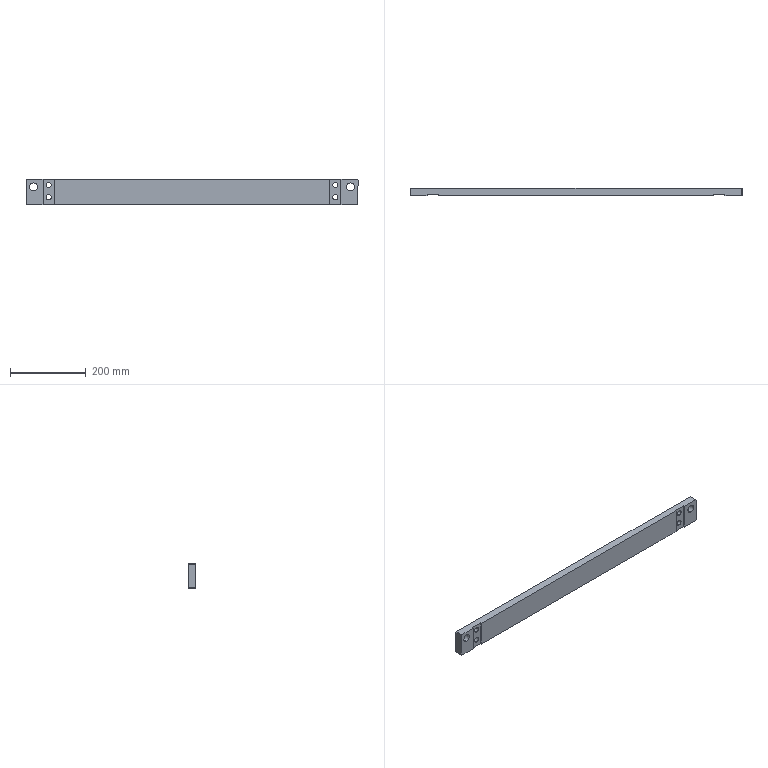Component | SolidWorks | FE2-211-_T_w_(-1 | 1 solid | 30 faces | box 878 x 20 x 67 mm | volume 1139978 mm3 | plane 18 | cylinder 12 | commonest cylinder face diameters 14 x8 21 x4
build123d program:
from build123d import *

# Parameters (mm, degrees)
SKETCH1_W      = 878
SKETCH1_H      = 67
EXTRUDE1_DEPTH = 20
SKETCH2_W      = 30
SKETCH2_H      = 67
EXTRUDE2_DEPTH = 3
SKETCH3_R      = 10.5
EXTRUDE3_DEPTH = 441.73
SKETCH4_R      = 7
EXTRUDE4_DEPTH = 441.604
CHAMFER1_SIZE  = 2


with BuildPart() as part:
    # Sketch1 → Extrude1 (new body)
    with BuildSketch(Plane(origin=(0, 0, 0), x_dir=(1, 0, 0), z_dir=(0, 1, 0))):
        Rectangle(SKETCH1_W, SKETCH1_H)
    extrude(amount=EXTRUDE1_DEPTH)

    # Sketch2 → Extrude2 (cut)
    with BuildSketch(Plane(origin=(0, 20, 0), x_dir=(1, 0, 0), z_dir=(0, 1, 0))):
        with Locations((379, 0)):
            Rectangle(SKETCH2_W, SKETCH2_H)
        with Locations((-379, 0)):
            Rectangle(SKETCH2_W, SKETCH2_H)
    extrude(amount=-EXTRUDE2_DEPTH, mode=Mode.SUBTRACT)

    # Sketch3 → Extrude3 (cut, through all)
    with BuildSketch(Plane(origin=(0, 20, 0), x_dir=(1, 0, 0), z_dir=(0, 1, 0))):
        with Locations(Location((419, 13.5, 0), (0, 0, 270))):
            Circle(SKETCH3_R)
        with Locations(Location((-419, 13.5, 0), (0, 0, 90))):
            Circle(SKETCH3_R)
    extrude(amount=-EXTRUDE3_DEPTH, mode=Mode.SUBTRACT)

    # Sketch4 → Extrude4 (cut, through all)
    with BuildSketch(Plane(origin=(0, 17, 0), x_dir=(1, 0, 0), z_dir=(0, 1, 0))):
        with Locations(Location((379, 18.5, 0), (0, 0, 270))):
            Circle(SKETCH4_R)
        with Locations(Location((379, -13.5, 0), (0, 0, 270))):
            Circle(SKETCH4_R)
        with Locations(Location((-379, -13.5, 0), (0, 0, 90))):
            Circle(SKETCH4_R)
        with Locations(Location((-379, 18.5, 0), (0, 0, 90))):
            Circle(SKETCH4_R)
    extrude(amount=-EXTRUDE4_DEPTH, mode=Mode.SUBTRACT)

    # Chamfer1
    chamfer1_edges = [part.edges().sort_by_distance(p)[0] for p in [
        (-439, 10, -33.5),
        (439, 10, -33.5),
        (439, 10, 33.5),
        (-439, 10, 33.5),
    ]]
    chamfer(chamfer1_edges, length=CHAMFER1_SIZE)


solid = part.part

# Placed as in the assembly
solid = solid.moved(Location((-379, 126.5, 311.5), (180, 0, 0)))
STEP:
#1=COLOUR_RGB('',0.7922,0.8196,0.9333);
#2=FILL_AREA_STYLE_COLOUR('',#1);
#3=FILL_AREA_STYLE('',(#2));
#4=SURFACE_STYLE_FILL_AREA(#3);
#5=SURFACE_SIDE_STYLE('',(#4));
#6=SURFACE_STYLE_USAGE(.BOTH.,#5);
#7=PRESENTATION_STYLE_ASSIGNMENT((#6));
#8=CARTESIAN_POINT('',(-29.843,4.98,13.268));
#9=VERTEX_POINT('',#8);
#10=CARTESIAN_POINT('',(-29.843,4.98,12.717));
#11=VERTEX_POINT('',#10);
#12=CARTESIAN_POINT('',(-29.843,4.98,12.992));
#13=DIRECTION('',(0.,-1.,0.));
#14=DIRECTION('',(0.,0.,1.));
#15=AXIS2_PLACEMENT_3D('',#12,#13,#14);
#16=CIRCLE('',#15,0.2756);
#17=EDGE_CURVE('',#9,#11,#16,.T.);
#18=ORIENTED_EDGE('',*,*,#17,.F.);
#19=CARTESIAN_POINT('',(-29.843,4.311,13.268));
#20=VERTEX_POINT('',#19);
#21=CARTESIAN_POINT('',(-29.843,4.98,13.268));
#22=DIRECTION('',(0.,-1.,0.));
#23=VECTOR('',#22,39.37);
#24=LINE('',#21,#23);
#25=EDGE_CURVE('',#9,#20,#24,.T.);
#26=ORIENTED_EDGE('',*,*,#25,.T.);
#27=CARTESIAN_POINT('',(-29.843,4.311,12.717));
#28=VERTEX_POINT('',#27);
#29=CARTESIAN_POINT('',(-29.843,4.311,12.992));
#30=DIRECTION('',(0.,-1.,0.));
#31=DIRECTION('',(0.,0.,1.));
#32=AXIS2_PLACEMENT_3D('',#29,#30,#31);
#33=CIRCLE('',#32,0.2756);
#34=EDGE_CURVE('',#20,#28,#33,.T.);
#35=ORIENTED_EDGE('',*,*,#34,.T.);
#36=CARTESIAN_POINT('',(-29.843,4.98,12.717));
#37=DIRECTION('',(0.,-1.,0.));
#38=VECTOR('',#37,39.37);
#39=LINE('',#36,#38);
#40=EDGE_CURVE('',#11,#28,#39,.T.);
#41=ORIENTED_EDGE('',*,*,#40,.F.);
#42=EDGE_LOOP('',(#18,#26,#35,#41));
#43=FACE_OUTER_BOUND('',#42,.T.);
#44=CARTESIAN_POINT('',(-29.843,4.98,12.992));
#45=DIRECTION('',(0.,-1.,0.));
#46=DIRECTION('',(0.,0.,-1.));
#47=AXIS2_PLACEMENT_3D('',#44,#45,#46);
#48=CYLINDRICAL_SURFACE('',#47,0.2756);
#49=ADVANCED_FACE('',(#43),#48,.F.);
#50=CARTESIAN_POINT('',(-29.843,4.98,12.008));
#51=VERTEX_POINT('',#50);
#52=CARTESIAN_POINT('',(-29.843,4.98,11.457));
#53=VERTEX_POINT('',#52);
#54=CARTESIAN_POINT('',(-29.843,4.98,11.732));
#55=DIRECTION('',(0.,-1.,0.));
#56=DIRECTION('',(0.,0.,1.));
#57=AXIS2_PLACEMENT_3D('',#54,#55,#56);
#58=CIRCLE('',#57,0.2756);
#59=EDGE_CURVE('',#51,#53,#58,.T.);
#60=ORIENTED_EDGE('',*,*,#59,.F.);
#61=CARTESIAN_POINT('',(-29.843,4.311,12.008));
#62=VERTEX_POINT('',#61);
#63=CARTESIAN_POINT('',(-29.843,4.98,12.008));
#64=DIRECTION('',(0.,-1.,0.));
#65=VECTOR('',#64,39.37);
#66=LINE('',#63,#65);
#67=EDGE_CURVE('',#51,#62,#66,.T.);
#68=ORIENTED_EDGE('',*,*,#67,.T.);
#69=CARTESIAN_POINT('',(-29.843,4.311,11.457));
#70=VERTEX_POINT('',#69);
#71=CARTESIAN_POINT('',(-29.843,4.311,11.732));
#72=DIRECTION('',(0.,-1.,0.));
#73=DIRECTION('',(0.,0.,1.));
#74=AXIS2_PLACEMENT_3D('',#71,#72,#73);
#75=CIRCLE('',#74,0.2756);
#76=EDGE_CURVE('',#62,#70,#75,.T.);
#77=ORIENTED_EDGE('',*,*,#76,.T.);
#78=CARTESIAN_POINT('',(-29.843,4.98,11.457));
#79=DIRECTION('',(0.,-1.,0.));
#80=VECTOR('',#79,39.37);
#81=LINE('',#78,#80);
#82=EDGE_CURVE('',#53,#70,#81,.T.);
#83=ORIENTED_EDGE('',*,*,#82,.F.);
#84=EDGE_LOOP('',(#60,#68,#77,#83));
#85=FACE_OUTER_BOUND('',#84,.T.);
#86=CARTESIAN_POINT('',(-29.843,4.98,11.732));
#87=DIRECTION('',(0.,-1.,0.));
#88=DIRECTION('',(0.,0.,-1.));
#89=AXIS2_PLACEMENT_3D('',#86,#87,#88);
#90=CYLINDRICAL_SURFACE('',#89,0.2756);
#91=ADVANCED_FACE('',(#85),#90,.F.);
#92=CARTESIAN_POINT('',(0.,4.98,12.008));
#93=VERTEX_POINT('',#92);
#94=CARTESIAN_POINT('',(0.,4.98,11.457));
#95=VERTEX_POINT('',#94);
#96=CARTESIAN_POINT('',(0.,4.98,11.732));
#97=DIRECTION('',(0.,-1.,0.));
#98=DIRECTION('',(-0.,0.,-1.));
#99=AXIS2_PLACEMENT_3D('',#96,#97,#98);
#100=CIRCLE('',#99,0.2756);
#101=EDGE_CURVE('',#93,#95,#100,.T.);
#102=ORIENTED_EDGE('',*,*,#101,.F.);
#103=CARTESIAN_POINT('',(0.,4.311,12.008));
#104=VERTEX_POINT('',#103);
#105=CARTESIAN_POINT('',(0.,4.98,12.008));
#106=DIRECTION('',(0.,-1.,0.));
#107=VECTOR('',#106,39.37);
#108=LINE('',#105,#107);
#109=EDGE_CURVE('',#93,#104,#108,.T.);
#110=ORIENTED_EDGE('',*,*,#109,.T.);
#111=CARTESIAN_POINT('',(0.,4.311,11.457));
#112=VERTEX_POINT('',#111);
#113=CARTESIAN_POINT('',(0.,4.311,11.732));
#114=DIRECTION('',(0.,-1.,0.));
#115=DIRECTION('',(-0.,0.,-1.));
#116=AXIS2_PLACEMENT_3D('',#113,#114,#115);
#117=CIRCLE('',#116,0.2756);
#118=EDGE_CURVE('',#104,#112,#117,.T.);
#119=ORIENTED_EDGE('',*,*,#118,.T.);
#120=CARTESIAN_POINT('',(0.,4.98,11.457));
#121=DIRECTION('',(0.,-1.,0.));
#122=VECTOR('',#121,39.37);
#123=LINE('',#120,#122);
#124=EDGE_CURVE('',#95,#112,#123,.T.);
#125=ORIENTED_EDGE('',*,*,#124,.F.);
#126=EDGE_LOOP('',(#102,#110,#119,#125));
#127=FACE_OUTER_BOUND('',#126,.T.);
#128=CARTESIAN_POINT('',(0.,4.98,11.732));
#129=DIRECTION('',(0.,-1.,0.));
#130=DIRECTION('',(-0.,0.,-1.));
#131=AXIS2_PLACEMENT_3D('',#128,#129,#130);
#132=CYLINDRICAL_SURFACE('',#131,0.2756);
#133=ADVANCED_FACE('',(#127),#132,.F.);
#134=CARTESIAN_POINT('',(0.,4.98,13.268));
#135=VERTEX_POINT('',#134);
#136=CARTESIAN_POINT('',(0.,4.98,12.717));
#137=VERTEX_POINT('',#136);
#138=CARTESIAN_POINT('',(0.,4.98,12.992));
#139=DIRECTION('',(0.,-1.,0.));
#140=DIRECTION('',(-0.,0.,-1.));
#141=AXIS2_PLACEMENT_3D('',#138,#139,#140);
#142=CIRCLE('',#141,0.2756);
#143=EDGE_CURVE('',#135,#137,#142,.T.);
#144=ORIENTED_EDGE('',*,*,#143,.F.);
#145=CARTESIAN_POINT('',(0.,4.311,13.268));
#146=VERTEX_POINT('',#145);
#147=CARTESIAN_POINT('',(0.,4.98,13.268));
#148=DIRECTION('',(0.,-1.,0.));
#149=VECTOR('',#148,39.37);
#150=LINE('',#147,#149);
#151=EDGE_CURVE('',#135,#146,#150,.T.);
#152=ORIENTED_EDGE('',*,*,#151,.T.);
#153=CARTESIAN_POINT('',(0.,4.311,12.717));
#154=VERTEX_POINT('',#153);
#155=CARTESIAN_POINT('',(0.,4.311,12.992));
#156=DIRECTION('',(0.,-1.,0.));
#157=DIRECTION('',(-0.,0.,-1.));
#158=AXIS2_PLACEMENT_3D('',#155,#156,#157);
#159=CIRCLE('',#158,0.2756);
#160=EDGE_CURVE('',#146,#154,#159,.T.);
#161=ORIENTED_EDGE('',*,*,#160,.T.);
#162=CARTESIAN_POINT('',(0.,4.98,12.717));
#163=DIRECTION('',(0.,-1.,0.));
#164=VECTOR('',#163,39.37);
#165=LINE('',#162,#164);
#166=EDGE_CURVE('',#137,#154,#165,.T.);
#167=ORIENTED_EDGE('',*,*,#166,.F.);
#168=EDGE_LOOP('',(#144,#152,#161,#167));
#169=FACE_OUTER_BOUND('',#168,.T.);
#170=CARTESIAN_POINT('',(0.,4.98,12.992));
#171=DIRECTION('',(0.,-1.,0.));
#172=DIRECTION('',(-0.,0.,-1.));
#173=AXIS2_PLACEMENT_3D('',#170,#171,#172);
#174=CYLINDRICAL_SURFACE('',#173,0.2756);
#175=ADVANCED_FACE('',(#169),#174,.F.);
#176=CARTESIAN_POINT('',(-31.417,4.98,13.209));
#177=VERTEX_POINT('',#176);
#178=CARTESIAN_POINT('',(-31.417,4.98,12.382));
#179=VERTEX_POINT('',#178);
#180=CARTESIAN_POINT('',(-31.417,4.98,12.795));
#181=DIRECTION('',(0.,-1.,0.));
#182=DIRECTION('',(0.,0.,1.));
#183=AXIS2_PLACEMENT_3D('',#180,#181,#182);
#184=CIRCLE('',#183,0.4134);
#185=EDGE_CURVE('',#177,#179,#184,.T.);
#186=ORIENTED_EDGE('',*,*,#185,.F.);
#187=CARTESIAN_POINT('',(-31.417,4.193,13.209));
#188=VERTEX_POINT('',#187);
#189=CARTESIAN_POINT('',(-31.417,4.98,13.209));
#190=DIRECTION('',(0.,-1.,0.));
#191=VECTOR('',#190,39.37);
#192=LINE('',#189,#191);
#193=EDGE_CURVE('',#177,#188,#192,.T.);
#194=ORIENTED_EDGE('',*,*,#193,.T.);
#195=CARTESIAN_POINT('',(-31.417,4.193,12.382));
#196=VERTEX_POINT('',#195);
#197=CARTESIAN_POINT('',(-31.417,4.193,12.795));
#198=DIRECTION('',(0.,-1.,0.));
#199=DIRECTION('',(0.,0.,1.));
#200=AXIS2_PLACEMENT_3D('',#197,#198,#199);
#201=CIRCLE('',#200,0.4134);
#202=EDGE_CURVE('',#188,#196,#201,.T.);
#203=ORIENTED_EDGE('',*,*,#202,.T.);
#204=CARTESIAN_POINT('',(-31.417,4.98,12.382));
#205=DIRECTION('',(0.,-1.,0.));
#206=VECTOR('',#205,39.37);
#207=LINE('',#204,#206);
#208=EDGE_CURVE('',#179,#196,#207,.T.);
#209=ORIENTED_EDGE('',*,*,#208,.F.);
#210=EDGE_LOOP('',(#186,#194,#203,#209));
#211=FACE_OUTER_BOUND('',#210,.T.);
#212=CARTESIAN_POINT('',(-31.417,4.98,12.795));
#213=DIRECTION('',(0.,-1.,0.));
#214=DIRECTION('',(0.,0.,-1.));
#215=AXIS2_PLACEMENT_3D('',#212,#213,#214);
#216=CYLINDRICAL_SURFACE('',#215,0.4134);
#217=ADVANCED_FACE('',(#211),#216,.F.);
#218=CARTESIAN_POINT('',(1.575,4.98,13.209));
#219=VERTEX_POINT('',#218);
#220=CARTESIAN_POINT('',(1.575,4.98,12.382));
#221=VERTEX_POINT('',#220);
#222=CARTESIAN_POINT('',(1.575,4.98,12.795));
#223=DIRECTION('',(0.,-1.,0.));
#224=DIRECTION('',(-0.,0.,-1.));
#225=AXIS2_PLACEMENT_3D('',#222,#223,#224);
#226=CIRCLE('',#225,0.4134);
#227=EDGE_CURVE('',#219,#221,#226,.T.);
#228=ORIENTED_EDGE('',*,*,#227,.F.);
#229=CARTESIAN_POINT('',(1.575,4.193,13.209));
#230=VERTEX_POINT('',#229);
#231=CARTESIAN_POINT('',(1.575,4.98,13.209));
#232=DIRECTION('',(0.,-1.,0.));
#233=VECTOR('',#232,39.37);
#234=LINE('',#231,#233);
#235=EDGE_CURVE('',#219,#230,#234,.T.);
#236=ORIENTED_EDGE('',*,*,#235,.T.);
#237=CARTESIAN_POINT('',(1.575,4.193,12.382));
#238=VERTEX_POINT('',#237);
#239=CARTESIAN_POINT('',(1.575,4.193,12.795));
#240=DIRECTION('',(0.,-1.,0.));
#241=DIRECTION('',(-0.,0.,-1.));
#242=AXIS2_PLACEMENT_3D('',#239,#240,#241);
#243=CIRCLE('',#242,0.4134);
#244=EDGE_CURVE('',#230,#238,#243,.T.);
#245=ORIENTED_EDGE('',*,*,#244,.T.);
#246=CARTESIAN_POINT('',(1.575,4.98,12.382));
#247=DIRECTION('',(0.,-1.,0.));
#248=VECTOR('',#247,39.37);
#249=LINE('',#246,#248);
#250=EDGE_CURVE('',#221,#238,#249,.T.);
#251=ORIENTED_EDGE('',*,*,#250,.F.);
#252=EDGE_LOOP('',(#228,#236,#245,#251));
#253=FACE_OUTER_BOUND('',#252,.T.);
#254=CARTESIAN_POINT('',(1.575,4.98,12.795));
#255=DIRECTION('',(0.,-1.,0.));
#256=DIRECTION('',(-0.,0.,-1.));
#257=AXIS2_PLACEMENT_3D('',#254,#255,#256);
#258=CYLINDRICAL_SURFACE('',#257,0.4134);
#259=ADVANCED_FACE('',(#253),#258,.F.);
#260=CARTESIAN_POINT('',(-29.252,4.193,10.945));
#261=VERTEX_POINT('',#260);
#262=CARTESIAN_POINT('',(-29.252,4.193,13.583));
#263=VERTEX_POINT('',#262);
#264=CARTESIAN_POINT('',(-29.252,4.193,13.583));
#265=DIRECTION('',(0.,0.,1.));
#266=VECTOR('',#265,39.37);
#267=LINE('',#264,#266);
#268=EDGE_CURVE('',#261,#263,#267,.T.);
#269=ORIENTED_EDGE('',*,*,#268,.F.);
#270=CARTESIAN_POINT('',(-0.5906,4.193,10.945));
#271=VERTEX_POINT('',#270);
#272=CARTESIAN_POINT('',(2.362,4.193,10.945));
#273=DIRECTION('',(1.,0.,-0.));
#274=VECTOR('',#273,39.37);
#275=LINE('',#272,#274);
#276=EDGE_CURVE('',#261,#271,#275,.T.);
#277=ORIENTED_EDGE('',*,*,#276,.T.);
#278=CARTESIAN_POINT('',(-0.5906,4.193,13.583));
#279=VERTEX_POINT('',#278);
#280=CARTESIAN_POINT('',(-0.5906,4.193,13.583));
#281=DIRECTION('',(-0.,0.,-1.));
#282=VECTOR('',#281,39.37);
#283=LINE('',#280,#282);
#284=EDGE_CURVE('',#279,#271,#283,.T.);
#285=ORIENTED_EDGE('',*,*,#284,.F.);
#286=CARTESIAN_POINT('',(2.362,4.193,13.583));
#287=DIRECTION('',(-1.,0.,0.));
#288=VECTOR('',#287,39.37);
#289=LINE('',#286,#288);
#290=EDGE_CURVE('',#279,#263,#289,.T.);
#291=ORIENTED_EDGE('',*,*,#290,.T.);
#292=EDGE_LOOP('',(#269,#277,#285,#291));
#293=FACE_OUTER_BOUND('',#292,.T.);
#294=CARTESIAN_POINT('',(-32.205,4.193,13.583));
#295=DIRECTION('',(0.,-1.,0.));
#296=DIRECTION('',(-0.,0.,-1.));
#297=AXIS2_PLACEMENT_3D('',#294,#295,#296);
#298=PLANE('',#297);
#299=ADVANCED_FACE('',(#293),#298,.T.);
#300=CARTESIAN_POINT('',(-31.417,4.193,12.795));
#301=DIRECTION('',(0.,-1.,0.));
#302=DIRECTION('',(0.,0.,1.));
#303=AXIS2_PLACEMENT_3D('',#300,#301,#302);
#304=CIRCLE('',#303,0.4134);
#305=EDGE_CURVE('',#196,#188,#304,.T.);
#306=ORIENTED_EDGE('',*,*,#305,.F.);
#307=ORIENTED_EDGE('',*,*,#202,.F.);
#308=EDGE_LOOP('',(#306,#307));
#309=FACE_BOUND('',#308,.T.);
#310=CARTESIAN_POINT('',(-30.433,4.193,13.583));
#311=VERTEX_POINT('',#310);
#312=CARTESIAN_POINT('',(-32.126,4.193,13.583));
#313=VERTEX_POINT('',#312);
#314=CARTESIAN_POINT('',(2.362,4.193,13.583));
#315=DIRECTION('',(-1.,0.,0.));
#316=VECTOR('',#315,39.37);
#317=LINE('',#314,#316);
#318=EDGE_CURVE('',#311,#313,#317,.T.);
#319=ORIENTED_EDGE('',*,*,#318,.T.);
#320=CARTESIAN_POINT('',(-32.205,4.193,13.504));
#321=VERTEX_POINT('',#320);
#322=CARTESIAN_POINT('',(-32.165,4.193,13.543));
#323=DIRECTION('',(-0.7071,0.,-0.7071));
#324=VECTOR('',#323,39.37);
#325=LINE('',#322,#324);
#326=EDGE_CURVE('',#313,#321,#325,.T.);
#327=ORIENTED_EDGE('',*,*,#326,.T.);
#328=CARTESIAN_POINT('',(-32.205,4.193,11.024));
#329=VERTEX_POINT('',#328);
#330=CARTESIAN_POINT('',(-32.205,4.193,10.945));
#331=DIRECTION('',(-0.,0.,-1.));
#332=VECTOR('',#331,39.37);
#333=LINE('',#330,#332);
#334=EDGE_CURVE('',#321,#329,#333,.T.);
#335=ORIENTED_EDGE('',*,*,#334,.T.);
#336=CARTESIAN_POINT('',(-32.126,4.193,10.945));
#337=VERTEX_POINT('',#336);
#338=CARTESIAN_POINT('',(-33.484,4.193,12.303));
#339=DIRECTION('',(0.7071,0.,-0.7071));
#340=VECTOR('',#339,39.37);
#341=LINE('',#338,#340);
#342=EDGE_CURVE('',#329,#337,#341,.T.);
#343=ORIENTED_EDGE('',*,*,#342,.T.);
#344=CARTESIAN_POINT('',(-30.433,4.193,10.945));
#345=VERTEX_POINT('',#344);
#346=CARTESIAN_POINT('',(2.362,4.193,10.945));
#347=DIRECTION('',(1.,0.,-0.));
#348=VECTOR('',#347,39.37);
#349=LINE('',#346,#348);
#350=EDGE_CURVE('',#337,#345,#349,.T.);
#351=ORIENTED_EDGE('',*,*,#350,.T.);
#352=CARTESIAN_POINT('',(-30.433,4.193,13.583));
#353=DIRECTION('',(-0.,0.,-1.));
#354=VECTOR('',#353,39.37);
#355=LINE('',#352,#354);
#356=EDGE_CURVE('',#311,#345,#355,.T.);
#357=ORIENTED_EDGE('',*,*,#356,.F.);
#358=EDGE_LOOP('',(#319,#327,#335,#343,#351,#357));
#359=FACE_OUTER_BOUND('',#358,.T.);
#360=CARTESIAN_POINT('',(-32.205,4.193,13.583));
#361=DIRECTION('',(0.,-1.,0.));
#362=DIRECTION('',(-0.,0.,-1.));
#363=AXIS2_PLACEMENT_3D('',#360,#361,#362);
#364=PLANE('',#363);
#365=ADVANCED_FACE('',(#309,#359),#364,.T.);
#366=ORIENTED_EDGE('',*,*,#334,.F.);
#367=CARTESIAN_POINT('',(-32.205,4.98,13.504));
#368=VERTEX_POINT('',#367);
#369=CARTESIAN_POINT('',(-32.205,4.193,13.504));
#370=DIRECTION('',(0.,1.,0.));
#371=VECTOR('',#370,39.37);
#372=LINE('',#369,#371);
#373=EDGE_CURVE('',#321,#368,#372,.T.);
#374=ORIENTED_EDGE('',*,*,#373,.T.);
#375=CARTESIAN_POINT('',(-32.205,4.98,11.024));
#376=VERTEX_POINT('',#375);
#377=CARTESIAN_POINT('',(-32.205,4.98,10.945));
#378=DIRECTION('',(-0.,0.,-1.));
#379=VECTOR('',#378,39.37);
#380=LINE('',#377,#379);
#381=EDGE_CURVE('',#368,#376,#380,.T.);
#382=ORIENTED_EDGE('',*,*,#381,.T.);
#383=CARTESIAN_POINT('',(-32.205,4.193,11.024));
#384=DIRECTION('',(0.,-1.,0.));
#385=VECTOR('',#384,39.37);
#386=LINE('',#383,#385);
#387=EDGE_CURVE('',#376,#329,#386,.T.);
#388=ORIENTED_EDGE('',*,*,#387,.T.);
#389=EDGE_LOOP('',(#366,#374,#382,#388));
#390=FACE_OUTER_BOUND('',#389,.T.);
#391=CARTESIAN_POINT('',(-32.205,4.193,10.945));
#392=DIRECTION('',(1.,0.,-0.));
#393=DIRECTION('',(0.,0.,1.));
#394=AXIS2_PLACEMENT_3D('',#391,#392,#393);
#395=PLANE('',#394);
#396=ADVANCED_FACE('',(#390),#395,.F.);
#397=CARTESIAN_POINT('',(-32.126,4.98,10.945));
#398=VERTEX_POINT('',#397);
#399=CARTESIAN_POINT('',(2.283,4.98,10.945));
#400=VERTEX_POINT('',#399);
#401=CARTESIAN_POINT('',(2.362,4.98,10.945));
#402=DIRECTION('',(1.,0.,-0.));
#403=VECTOR('',#402,39.37);
#404=LINE('',#401,#403);
#405=EDGE_CURVE('',#398,#400,#404,.T.);
#406=ORIENTED_EDGE('',*,*,#405,.T.);
#407=CARTESIAN_POINT('',(2.283,4.193,10.945));
#408=VERTEX_POINT('',#407);
#409=CARTESIAN_POINT('',(2.283,4.193,10.945));
#410=DIRECTION('',(0.,-1.,0.));
#411=VECTOR('',#410,39.37);
#412=LINE('',#409,#411);
#413=EDGE_CURVE('',#400,#408,#412,.T.);
#414=ORIENTED_EDGE('',*,*,#413,.T.);
#415=CARTESIAN_POINT('',(0.5906,4.193,10.945));
#416=VERTEX_POINT('',#415);
#417=CARTESIAN_POINT('',(2.362,4.193,10.945));
#418=DIRECTION('',(1.,0.,-0.));
#419=VECTOR('',#418,39.37);
#420=LINE('',#417,#419);
#421=EDGE_CURVE('',#416,#408,#420,.T.);
#422=ORIENTED_EDGE('',*,*,#421,.F.);
#423=CARTESIAN_POINT('',(0.5906,4.311,10.945));
#424=VERTEX_POINT('',#423);
#425=CARTESIAN_POINT('',(0.5906,4.311,10.945));
#426=DIRECTION('',(0.,-1.,0.));
#427=VECTOR('',#426,39.37);
#428=LINE('',#425,#427);
#429=EDGE_CURVE('',#424,#416,#428,.T.);
#430=ORIENTED_EDGE('',*,*,#429,.F.);
#431=CARTESIAN_POINT('',(-0.5906,4.311,10.945));
#432=VERTEX_POINT('',#431);
#433=CARTESIAN_POINT('',(-0.5906,4.311,10.945));
#434=DIRECTION('',(1.,0.,-0.));
#435=VECTOR('',#434,39.37);
#436=LINE('',#433,#435);
#437=EDGE_CURVE('',#432,#424,#436,.T.);
#438=ORIENTED_EDGE('',*,*,#437,.F.);
#439=CARTESIAN_POINT('',(-0.5906,4.311,10.945));
#440=DIRECTION('',(0.,-1.,0.));
#441=VECTOR('',#440,39.37);
#442=LINE('',#439,#441);
#443=EDGE_CURVE('',#432,#271,#442,.T.);
#444=ORIENTED_EDGE('',*,*,#443,.T.);
#445=ORIENTED_EDGE('',*,*,#276,.F.);
#446=CARTESIAN_POINT('',(-29.252,4.311,10.945));
#447=VERTEX_POINT('',#446);
#448=CARTESIAN_POINT('',(-29.252,4.311,10.945));
#449=DIRECTION('',(0.,-1.,0.));
#450=VECTOR('',#449,39.37);
#451=LINE('',#448,#450);
#452=EDGE_CURVE('',#447,#261,#451,.T.);
#453=ORIENTED_EDGE('',*,*,#452,.F.);
#454=CARTESIAN_POINT('',(-30.433,4.311,10.945));
#455=VERTEX_POINT('',#454);
#456=CARTESIAN_POINT('',(-29.252,4.311,10.945));
#457=DIRECTION('',(1.,0.,-0.));
#458=VECTOR('',#457,39.37);
#459=LINE('',#456,#458);
#460=EDGE_CURVE('',#455,#447,#459,.T.);
#461=ORIENTED_EDGE('',*,*,#460,.F.);
#462=CARTESIAN_POINT('',(-30.433,4.311,10.945));
#463=DIRECTION('',(0.,-1.,0.));
#464=VECTOR('',#463,39.37);
#465=LINE('',#462,#464);
#466=EDGE_CURVE('',#455,#345,#465,.T.);
#467=ORIENTED_EDGE('',*,*,#466,.T.);
#468=ORIENTED_EDGE('',*,*,#350,.F.);
#469=CARTESIAN_POINT('',(-32.126,4.193,10.945));
#470=DIRECTION('',(0.,1.,0.));
#471=VECTOR('',#470,39.37);
#472=LINE('',#469,#471);
#473=EDGE_CURVE('',#337,#398,#472,.T.);
#474=ORIENTED_EDGE('',*,*,#473,.T.);
#475=EDGE_LOOP('',(#406,#414,#422,#430,#438,#444,#445,#453,#461,#467,#468,#474));
#476=FACE_OUTER_BOUND('',#475,.T.);
#477=CARTESIAN_POINT('',(2.362,4.193,10.945));
#478=DIRECTION('',(0.,0.,1.));
#479=DIRECTION('',(-1.,0.,0.));
#480=AXIS2_PLACEMENT_3D('',#477,#478,#479);
#481=PLANE('',#480);
#482=ADVANCED_FACE('',(#476),#481,.F.);
#483=CARTESIAN_POINT('',(2.362,4.98,11.024));
#484=VERTEX_POINT('',#483);
#485=CARTESIAN_POINT('',(2.362,4.98,13.504));
#486=VERTEX_POINT('',#485);
#487=CARTESIAN_POINT('',(2.362,4.98,10.945));
#488=DIRECTION('',(0.,0.,1.));
#489=VECTOR('',#488,39.37);
#490=LINE('',#487,#489);
#491=EDGE_CURVE('',#484,#486,#490,.T.);
#492=ORIENTED_EDGE('',*,*,#491,.T.);
#493=CARTESIAN_POINT('',(2.362,4.193,13.504));
#494=VERTEX_POINT('',#493);
#495=CARTESIAN_POINT('',(2.362,4.193,13.504));
#496=DIRECTION('',(0.,-1.,0.));
#497=VECTOR('',#496,39.37);
#498=LINE('',#495,#497);
#499=EDGE_CURVE('',#486,#494,#498,.T.);
#500=ORIENTED_EDGE('',*,*,#499,.T.);
#501=CARTESIAN_POINT('',(2.362,4.193,11.024));
#502=VERTEX_POINT('',#501);
#503=CARTESIAN_POINT('',(2.362,4.193,10.945));
#504=DIRECTION('',(0.,0.,1.));
#505=VECTOR('',#504,39.37);
#506=LINE('',#503,#505);
#507=EDGE_CURVE('',#502,#494,#506,.T.);
#508=ORIENTED_EDGE('',*,*,#507,.F.);
#509=CARTESIAN_POINT('',(2.362,4.193,11.024));
#510=DIRECTION('',(0.,1.,0.));
#511=VECTOR('',#510,39.37);
#512=LINE('',#509,#511);
#513=EDGE_CURVE('',#502,#484,#512,.T.);
#514=ORIENTED_EDGE('',*,*,#513,.T.);
#515=EDGE_LOOP('',(#492,#500,#508,#514));
#516=FACE_OUTER_BOUND('',#515,.T.);
#517=CARTESIAN_POINT('',(2.362,4.193,10.945));
#518=DIRECTION('',(-1.,0.,0.));
#519=DIRECTION('',(-0.,0.,-1.));
#520=AXIS2_PLACEMENT_3D('',#517,#518,#519);
#521=PLANE('',#520);
#522=ADVANCED_FACE('',(#516),#521,.F.);
#523=CARTESIAN_POINT('',(2.283,4.193,13.583));
#524=VERTEX_POINT('',#523);
#525=CARTESIAN_POINT('',(0.5906,4.193,13.583));
#526=VERTEX_POINT('',#525);
#527=CARTESIAN_POINT('',(2.362,4.193,13.583));
#528=DIRECTION('',(-1.,0.,0.));
#529=VECTOR('',#528,39.37);
#530=LINE('',#527,#529);
#531=EDGE_CURVE('',#524,#526,#530,.T.);
#532=ORIENTED_EDGE('',*,*,#531,.F.);
#533=CARTESIAN_POINT('',(2.283,4.98,13.583));
#534=VERTEX_POINT('',#533);
#535=CARTESIAN_POINT('',(2.283,4.193,13.583));
#536=DIRECTION('',(0.,1.,0.));
#537=VECTOR('',#536,39.37);
#538=LINE('',#535,#537);
#539=EDGE_CURVE('',#524,#534,#538,.T.);
#540=ORIENTED_EDGE('',*,*,#539,.T.);
#541=CARTESIAN_POINT('',(-32.126,4.98,13.583));
#542=VERTEX_POINT('',#541);
#543=CARTESIAN_POINT('',(2.362,4.98,13.583));
#544=DIRECTION('',(-1.,0.,0.));
#545=VECTOR('',#544,39.37);
#546=LINE('',#543,#545);
#547=EDGE_CURVE('',#534,#542,#546,.T.);
#548=ORIENTED_EDGE('',*,*,#547,.T.);
#549=CARTESIAN_POINT('',(-32.126,4.193,13.583));
#550=DIRECTION('',(0.,-1.,0.));
#551=VECTOR('',#550,39.37);
#552=LINE('',#549,#551);
#553=EDGE_CURVE('',#542,#313,#552,.T.);
#554=ORIENTED_EDGE('',*,*,#553,.T.);
#555=ORIENTED_EDGE('',*,*,#318,.F.);
#556=CARTESIAN_POINT('',(-30.433,4.311,13.583));
#557=VERTEX_POINT('',#556);
#558=CARTESIAN_POINT('',(-30.433,4.311,13.583));
#559=DIRECTION('',(0.,-1.,0.));
#560=VECTOR('',#559,39.37);
#561=LINE('',#558,#560);
#562=EDGE_CURVE('',#557,#311,#561,.T.);
#563=ORIENTED_EDGE('',*,*,#562,.F.);
#564=CARTESIAN_POINT('',(-29.252,4.311,13.583));
#565=VERTEX_POINT('',#564);
#566=CARTESIAN_POINT('',(-29.252,4.311,13.583));
#567=DIRECTION('',(-1.,0.,0.));
#568=VECTOR('',#567,39.37);
#569=LINE('',#566,#568);
#570=EDGE_CURVE('',#565,#557,#569,.T.);
#571=ORIENTED_EDGE('',*,*,#570,.F.);
#572=CARTESIAN_POINT('',(-29.252,4.311,13.583));
#573=DIRECTION('',(0.,-1.,0.));
#574=VECTOR('',#573,39.37);
#575=LINE('',#572,#574);
#576=EDGE_CURVE('',#565,#263,#575,.T.);
#577=ORIENTED_EDGE('',*,*,#576,.T.);
#578=ORIENTED_EDGE('',*,*,#290,.F.);
#579=CARTESIAN_POINT('',(-0.5906,4.311,13.583));
#580=VERTEX_POINT('',#579);
#581=CARTESIAN_POINT('',(-0.5906,4.311,13.583));
#582=DIRECTION('',(0.,-1.,0.));
#583=VECTOR('',#582,39.37);
#584=LINE('',#581,#583);
#585=EDGE_CURVE('',#580,#279,#584,.T.);
#586=ORIENTED_EDGE('',*,*,#585,.F.);
#587=CARTESIAN_POINT('',(0.5906,4.311,13.583));
#588=VERTEX_POINT('',#587);
#589=CARTESIAN_POINT('',(-0.5906,4.311,13.583));
#590=DIRECTION('',(-1.,0.,0.));
#591=VECTOR('',#590,39.37);
#592=LINE('',#589,#591);
#593=EDGE_CURVE('',#588,#580,#592,.T.);
#594=ORIENTED_EDGE('',*,*,#593,.F.);
#595=CARTESIAN_POINT('',(0.5906,4.311,13.583));
#596=DIRECTION('',(0.,-1.,0.));
#597=VECTOR('',#596,39.37);
#598=LINE('',#595,#597);
#599=EDGE_CURVE('',#588,#526,#598,.T.);
#600=ORIENTED_EDGE('',*,*,#599,.T.);
#601=EDGE_LOOP('',(#532,#540,#548,#554,#555,#563,#571,#577,#578,#586,#594,#600));
#602=FACE_OUTER_BOUND('',#601,.T.);
#603=CARTESIAN_POINT('',(2.362,4.193,13.583));
#604=DIRECTION('',(-0.,0.,-1.));
#605=DIRECTION('',(1.,0.,-0.));
#606=AXIS2_PLACEMENT_3D('',#603,#604,#605);
#607=PLANE('',#606);
#608=ADVANCED_FACE('',(#602),#607,.F.);
#609=CARTESIAN_POINT('',(1.575,4.193,12.795));
#610=DIRECTION('',(0.,-1.,0.));
#611=DIRECTION('',(-0.,0.,-1.));
#612=AXIS2_PLACEMENT_3D('',#609,#610,#611);
#613=CIRCLE('',#612,0.4134);
#614=EDGE_CURVE('',#238,#230,#613,.T.);
#615=ORIENTED_EDGE('',*,*,#614,.F.);
#616=ORIENTED_EDGE('',*,*,#244,.F.);
#617=EDGE_LOOP('',(#615,#616));
#618=FACE_BOUND('',#617,.T.);
#619=ORIENTED_EDGE('',*,*,#507,.T.);
#620=CARTESIAN_POINT('',(-14.961,4.193,30.827));
#621=DIRECTION('',(-0.7071,0.,0.7071));
#622=VECTOR('',#621,39.37);
#623=LINE('',#620,#622);
#624=EDGE_CURVE('',#494,#524,#623,.T.);
#625=ORIENTED_EDGE('',*,*,#624,.T.);
#626=ORIENTED_EDGE('',*,*,#531,.T.);
#627=CARTESIAN_POINT('',(0.5906,4.193,13.583));
#628=DIRECTION('',(0.,0.,1.));
#629=VECTOR('',#628,39.37);
#630=LINE('',#627,#629);
#631=EDGE_CURVE('',#416,#526,#630,.T.);
#632=ORIENTED_EDGE('',*,*,#631,.F.);
#633=ORIENTED_EDGE('',*,*,#421,.T.);
#634=CARTESIAN_POINT('',(-13.642,4.193,-4.98));
#635=DIRECTION('',(0.7071,0.,0.7071));
#636=VECTOR('',#635,39.37);
#637=LINE('',#634,#636);
#638=EDGE_CURVE('',#408,#502,#637,.T.);
#639=ORIENTED_EDGE('',*,*,#638,.T.);
#640=EDGE_LOOP('',(#619,#625,#626,#632,#633,#639));
#641=FACE_OUTER_BOUND('',#640,.T.);
#642=CARTESIAN_POINT('',(-32.205,4.193,13.583));
#643=DIRECTION('',(0.,-1.,0.));
#644=DIRECTION('',(-0.,0.,-1.));
#645=AXIS2_PLACEMENT_3D('',#642,#643,#644);
#646=PLANE('',#645);
#647=ADVANCED_FACE('',(#618,#641),#646,.T.);
#648=CARTESIAN_POINT('',(-29.843,4.98,12.992));
#649=DIRECTION('',(0.,-1.,0.));
#650=DIRECTION('',(0.,0.,1.));
#651=AXIS2_PLACEMENT_3D('',#648,#649,#650);
#652=CIRCLE('',#651,0.2756);
#653=EDGE_CURVE('',#11,#9,#652,.T.);
#654=ORIENTED_EDGE('',*,*,#653,.T.);
#655=ORIENTED_EDGE('',*,*,#17,.T.);
#656=EDGE_LOOP('',(#654,#655));
#657=FACE_BOUND('',#656,.T.);
#658=CARTESIAN_POINT('',(-29.843,4.98,11.732));
#659=DIRECTION('',(0.,-1.,0.));
#660=DIRECTION('',(0.,0.,1.));
#661=AXIS2_PLACEMENT_3D('',#658,#659,#660);
#662=CIRCLE('',#661,0.2756);
#663=EDGE_CURVE('',#53,#51,#662,.T.);
#664=ORIENTED_EDGE('',*,*,#663,.T.);
#665=ORIENTED_EDGE('',*,*,#59,.T.);
#666=EDGE_LOOP('',(#664,#665));
#667=FACE_BOUND('',#666,.T.);
#668=CARTESIAN_POINT('',(0.,4.98,11.732));
#669=DIRECTION('',(0.,-1.,0.));
#670=DIRECTION('',(-0.,0.,-1.));
#671=AXIS2_PLACEMENT_3D('',#668,#669,#670);
#672=CIRCLE('',#671,0.2756);
#673=EDGE_CURVE('',#95,#93,#672,.T.);
#674=ORIENTED_EDGE('',*,*,#673,.T.);
#675=ORIENTED_EDGE('',*,*,#101,.T.);
#676=EDGE_LOOP('',(#674,#675));
#677=FACE_BOUND('',#676,.T.);
#678=CARTESIAN_POINT('',(0.,4.98,12.992));
#679=DIRECTION('',(0.,-1.,0.));
#680=DIRECTION('',(-0.,0.,-1.));
#681=AXIS2_PLACEMENT_3D('',#678,#679,#680);
#682=CIRCLE('',#681,0.2756);
#683=EDGE_CURVE('',#137,#135,#682,.T.);
#684=ORIENTED_EDGE('',*,*,#683,.T.);
#685=ORIENTED_EDGE('',*,*,#143,.T.);
#686=EDGE_LOOP('',(#684,#685));
#687=FACE_BOUND('',#686,.T.);
#688=CARTESIAN_POINT('',(-31.417,4.98,12.795));
#689=DIRECTION('',(0.,-1.,0.));
#690=DIRECTION('',(0.,0.,1.));
#691=AXIS2_PLACEMENT_3D('',#688,#689,#690);
#692=CIRCLE('',#691,0.4134);
#693=EDGE_CURVE('',#179,#177,#692,.T.);
#694=ORIENTED_EDGE('',*,*,#693,.T.);
#695=ORIENTED_EDGE('',*,*,#185,.T.);
#696=EDGE_LOOP('',(#694,#695));
#697=FACE_BOUND('',#696,.T.);
#698=CARTESIAN_POINT('',(1.575,4.98,12.795));
#699=DIRECTION('',(0.,-1.,0.));
#700=DIRECTION('',(-0.,0.,-1.));
#701=AXIS2_PLACEMENT_3D('',#698,#699,#700);
#702=CIRCLE('',#701,0.4134);
#703=EDGE_CURVE('',#221,#219,#702,.T.);
#704=ORIENTED_EDGE('',*,*,#703,.T.);
#705=ORIENTED_EDGE('',*,*,#227,.T.);
#706=EDGE_LOOP('',(#704,#705));
#707=FACE_BOUND('',#706,.T.);
#708=ORIENTED_EDGE('',*,*,#547,.F.);
#709=CARTESIAN_POINT('',(2.283,4.98,13.583));
#710=DIRECTION('',(0.7071,0.,-0.7071));
#711=VECTOR('',#710,39.37);
#712=LINE('',#709,#711);
#713=EDGE_CURVE('',#534,#486,#712,.T.);
#714=ORIENTED_EDGE('',*,*,#713,.T.);
#715=ORIENTED_EDGE('',*,*,#491,.F.);
#716=CARTESIAN_POINT('',(2.362,4.98,11.024));
#717=DIRECTION('',(-0.7071,0.,-0.7071));
#718=VECTOR('',#717,39.37);
#719=LINE('',#716,#718);
#720=EDGE_CURVE('',#484,#400,#719,.T.);
#721=ORIENTED_EDGE('',*,*,#720,.T.);
#722=ORIENTED_EDGE('',*,*,#405,.F.);
#723=CARTESIAN_POINT('',(-32.126,4.98,10.945));
#724=DIRECTION('',(-0.7071,0.,0.7071));
#725=VECTOR('',#724,39.37);
#726=LINE('',#723,#725);
#727=EDGE_CURVE('',#398,#376,#726,.T.);
#728=ORIENTED_EDGE('',*,*,#727,.T.);
#729=ORIENTED_EDGE('',*,*,#381,.F.);
#730=CARTESIAN_POINT('',(-32.205,4.98,13.504));
#731=DIRECTION('',(0.7071,0.,0.7071));
#732=VECTOR('',#731,39.37);
#733=LINE('',#730,#732);
#734=EDGE_CURVE('',#368,#542,#733,.T.);
#735=ORIENTED_EDGE('',*,*,#734,.T.);
#736=EDGE_LOOP('',(#708,#714,#715,#721,#722,#728,#729,#735));
#737=FACE_OUTER_BOUND('',#736,.T.);
#738=CARTESIAN_POINT('',(-32.205,4.98,13.583));
#739=DIRECTION('',(0.,-1.,0.));
#740=DIRECTION('',(-0.,0.,-1.));
#741=AXIS2_PLACEMENT_3D('',#738,#739,#740);
#742=PLANE('',#741);
#743=ADVANCED_FACE('',(#657,#667,#677,#687,#697,#707,#737),#742,.F.);
#744=ORIENTED_EDGE('',*,*,#284,.T.);
#745=ORIENTED_EDGE('',*,*,#443,.F.);
#746=CARTESIAN_POINT('',(-0.5906,4.311,13.583));
#747=DIRECTION('',(-0.,0.,-1.));
#748=VECTOR('',#747,39.37);
#749=LINE('',#746,#748);
#750=EDGE_CURVE('',#580,#432,#749,.T.);
#751=ORIENTED_EDGE('',*,*,#750,.F.);
#752=ORIENTED_EDGE('',*,*,#585,.T.);
#753=EDGE_LOOP('',(#744,#745,#751,#752));
#754=FACE_OUTER_BOUND('',#753,.T.);
#755=CARTESIAN_POINT('',(-0.5906,4.311,13.583));
#756=DIRECTION('',(-1.,0.,0.));
#757=DIRECTION('',(-0.,0.,-1.));
#758=AXIS2_PLACEMENT_3D('',#755,#756,#757);
#759=PLANE('',#758);
#760=ADVANCED_FACE('',(#754),#759,.F.);
#761=ORIENTED_EDGE('',*,*,#631,.T.);
#762=ORIENTED_EDGE('',*,*,#599,.F.);
#763=CARTESIAN_POINT('',(0.5906,4.311,13.583));
#764=DIRECTION('',(0.,0.,1.));
#765=VECTOR('',#764,39.37);
#766=LINE('',#763,#765);
#767=EDGE_CURVE('',#424,#588,#766,.T.);
#768=ORIENTED_EDGE('',*,*,#767,.F.);
#769=ORIENTED_EDGE('',*,*,#429,.T.);
#770=EDGE_LOOP('',(#761,#762,#768,#769));
#771=FACE_OUTER_BOUND('',#770,.T.);
#772=CARTESIAN_POINT('',(0.5906,4.311,13.583));
#773=DIRECTION('',(1.,0.,-0.));
#774=DIRECTION('',(0.,0.,1.));
#775=AXIS2_PLACEMENT_3D('',#772,#773,#774);
#776=PLANE('',#775);
#777=ADVANCED_FACE('',(#771),#776,.F.);
#778=CARTESIAN_POINT('',(0.,4.311,11.732));
#779=DIRECTION('',(0.,-1.,0.));
#780=DIRECTION('',(-0.,0.,-1.));
#781=AXIS2_PLACEMENT_3D('',#778,#779,#780);
#782=CIRCLE('',#781,0.2756);
#783=EDGE_CURVE('',#112,#104,#782,.T.);
#784=ORIENTED_EDGE('',*,*,#783,.F.);
#785=ORIENTED_EDGE('',*,*,#118,.F.);
#786=EDGE_LOOP('',(#784,#785));
#787=FACE_BOUND('',#786,.T.);
#788=CARTESIAN_POINT('',(0.,4.311,12.992));
#789=DIRECTION('',(0.,-1.,0.));
#790=DIRECTION('',(-0.,0.,-1.));
#791=AXIS2_PLACEMENT_3D('',#788,#789,#790);
#792=CIRCLE('',#791,0.2756);
#793=EDGE_CURVE('',#154,#146,#792,.T.);
#794=ORIENTED_EDGE('',*,*,#793,.F.);
#795=ORIENTED_EDGE('',*,*,#160,.F.);
#796=EDGE_LOOP('',(#794,#795));
#797=FACE_BOUND('',#796,.T.);
#798=ORIENTED_EDGE('',*,*,#750,.T.);
#799=ORIENTED_EDGE('',*,*,#437,.T.);
#800=ORIENTED_EDGE('',*,*,#767,.T.);
#801=ORIENTED_EDGE('',*,*,#593,.T.);
#802=EDGE_LOOP('',(#798,#799,#800,#801));
#803=FACE_OUTER_BOUND('',#802,.T.);
#804=CARTESIAN_POINT('',(-0.5906,4.311,10.945));
#805=DIRECTION('',(0.,-1.,0.));
#806=DIRECTION('',(-0.,0.,-1.));
#807=AXIS2_PLACEMENT_3D('',#804,#805,#806);
#808=PLANE('',#807);
#809=ADVANCED_FACE('',(#787,#797,#803),#808,.T.);
#810=ORIENTED_EDGE('',*,*,#268,.T.);
#811=ORIENTED_EDGE('',*,*,#576,.F.);
#812=CARTESIAN_POINT('',(-29.252,4.311,13.583));
#813=DIRECTION('',(0.,0.,1.));
#814=VECTOR('',#813,39.37);
#815=LINE('',#812,#814);
#816=EDGE_CURVE('',#447,#565,#815,.T.);
#817=ORIENTED_EDGE('',*,*,#816,.F.);
#818=ORIENTED_EDGE('',*,*,#452,.T.);
#819=EDGE_LOOP('',(#810,#811,#817,#818));
#820=FACE_OUTER_BOUND('',#819,.T.);
#821=CARTESIAN_POINT('',(-29.252,4.311,13.583));
#822=DIRECTION('',(1.,0.,-0.));
#823=DIRECTION('',(0.,0.,1.));
#824=AXIS2_PLACEMENT_3D('',#821,#822,#823);
#825=PLANE('',#824);
#826=ADVANCED_FACE('',(#820),#825,.F.);
#827=ORIENTED_EDGE('',*,*,#356,.T.);
#828=ORIENTED_EDGE('',*,*,#466,.F.);
#829=CARTESIAN_POINT('',(-30.433,4.311,13.583));
#830=DIRECTION('',(-0.,0.,-1.));
#831=VECTOR('',#830,39.37);
#832=LINE('',#829,#831);
#833=EDGE_CURVE('',#557,#455,#832,.T.);
#834=ORIENTED_EDGE('',*,*,#833,.F.);
#835=ORIENTED_EDGE('',*,*,#562,.T.);
#836=EDGE_LOOP('',(#827,#828,#834,#835));
#837=FACE_OUTER_BOUND('',#836,.T.);
#838=CARTESIAN_POINT('',(-30.433,4.311,13.583));
#839=DIRECTION('',(-1.,0.,0.));
#840=DIRECTION('',(-0.,0.,-1.));
#841=AXIS2_PLACEMENT_3D('',#838,#839,#840);
#842=PLANE('',#841);
#843=ADVANCED_FACE('',(#837),#842,.F.);
#844=CARTESIAN_POINT('',(-29.843,4.311,12.992));
#845=DIRECTION('',(0.,-1.,0.));
#846=DIRECTION('',(0.,0.,1.));
#847=AXIS2_PLACEMENT_3D('',#844,#845,#846);
#848=CIRCLE('',#847,0.2756);
#849=EDGE_CURVE('',#28,#20,#848,.T.);
#850=ORIENTED_EDGE('',*,*,#849,.F.);
#851=ORIENTED_EDGE('',*,*,#34,.F.);
#852=EDGE_LOOP('',(#850,#851));
#853=FACE_BOUND('',#852,.T.);
#854=CARTESIAN_POINT('',(-29.843,4.311,11.732));
#855=DIRECTION('',(0.,-1.,0.));
#856=DIRECTION('',(0.,0.,1.));
#857=AXIS2_PLACEMENT_3D('',#854,#855,#856);
#858=CIRCLE('',#857,0.2756);
#859=EDGE_CURVE('',#70,#62,#858,.T.);
#860=ORIENTED_EDGE('',*,*,#859,.F.);
#861=ORIENTED_EDGE('',*,*,#76,.F.);
#862=EDGE_LOOP('',(#860,#861));
#863=FACE_BOUND('',#862,.T.);
#864=ORIENTED_EDGE('',*,*,#570,.T.);
#865=ORIENTED_EDGE('',*,*,#833,.T.);
#866=ORIENTED_EDGE('',*,*,#460,.T.);
#867=ORIENTED_EDGE('',*,*,#816,.T.);
#868=EDGE_LOOP('',(#864,#865,#866,#867));
#869=FACE_OUTER_BOUND('',#868,.T.);
#870=CARTESIAN_POINT('',(-30.433,4.311,13.583));
#871=DIRECTION('',(0.,-1.,0.));
#872=DIRECTION('',(-0.,0.,-1.));
#873=AXIS2_PLACEMENT_3D('',#870,#871,#872);
#874=PLANE('',#873);
#875=ADVANCED_FACE('',(#853,#863,#869),#874,.T.);
#876=ORIENTED_EDGE('',*,*,#235,.F.);
#877=ORIENTED_EDGE('',*,*,#703,.F.);
#878=ORIENTED_EDGE('',*,*,#250,.T.);
#879=ORIENTED_EDGE('',*,*,#614,.T.);
#880=EDGE_LOOP('',(#876,#877,#878,#879));
#881=FACE_OUTER_BOUND('',#880,.T.);
#882=CARTESIAN_POINT('',(1.575,4.98,12.795));
#883=DIRECTION('',(0.,-1.,0.));
#884=DIRECTION('',(-0.,0.,-1.));
#885=AXIS2_PLACEMENT_3D('',#882,#883,#884);
#886=CYLINDRICAL_SURFACE('',#885,0.4134);
#887=ADVANCED_FACE('',(#881),#886,.F.);
#888=ORIENTED_EDGE('',*,*,#193,.F.);
#889=ORIENTED_EDGE('',*,*,#693,.F.);
#890=ORIENTED_EDGE('',*,*,#208,.T.);
#891=ORIENTED_EDGE('',*,*,#305,.T.);
#892=EDGE_LOOP('',(#888,#889,#890,#891));
#893=FACE_OUTER_BOUND('',#892,.T.);
#894=CARTESIAN_POINT('',(-31.417,4.98,12.795));
#895=DIRECTION('',(0.,-1.,0.));
#896=DIRECTION('',(0.,0.,-1.));
#897=AXIS2_PLACEMENT_3D('',#894,#895,#896);
#898=CYLINDRICAL_SURFACE('',#897,0.4134);
#899=ADVANCED_FACE('',(#893),#898,.F.);
#900=ORIENTED_EDGE('',*,*,#151,.F.);
#901=ORIENTED_EDGE('',*,*,#683,.F.);
#902=ORIENTED_EDGE('',*,*,#166,.T.);
#903=ORIENTED_EDGE('',*,*,#793,.T.);
#904=EDGE_LOOP('',(#900,#901,#902,#903));
#905=FACE_OUTER_BOUND('',#904,.T.);
#906=CARTESIAN_POINT('',(0.,4.98,12.992));
#907=DIRECTION('',(0.,-1.,0.));
#908=DIRECTION('',(-0.,0.,-1.));
#909=AXIS2_PLACEMENT_3D('',#906,#907,#908);
#910=CYLINDRICAL_SURFACE('',#909,0.2756);
#911=ADVANCED_FACE('',(#905),#910,.F.);
#912=ORIENTED_EDGE('',*,*,#109,.F.);
#913=ORIENTED_EDGE('',*,*,#673,.F.);
#914=ORIENTED_EDGE('',*,*,#124,.T.);
#915=ORIENTED_EDGE('',*,*,#783,.T.);
#916=EDGE_LOOP('',(#912,#913,#914,#915));
#917=FACE_OUTER_BOUND('',#916,.T.);
#918=CARTESIAN_POINT('',(0.,4.98,11.732));
#919=DIRECTION('',(0.,-1.,0.));
#920=DIRECTION('',(-0.,0.,-1.));
#921=AXIS2_PLACEMENT_3D('',#918,#919,#920);
#922=CYLINDRICAL_SURFACE('',#921,0.2756);
#923=ADVANCED_FACE('',(#917),#922,.F.);
#924=ORIENTED_EDGE('',*,*,#67,.F.);
#925=ORIENTED_EDGE('',*,*,#663,.F.);
#926=ORIENTED_EDGE('',*,*,#82,.T.);
#927=ORIENTED_EDGE('',*,*,#859,.T.);
#928=EDGE_LOOP('',(#924,#925,#926,#927));
#929=FACE_OUTER_BOUND('',#928,.T.);
#930=CARTESIAN_POINT('',(-29.843,4.98,11.732));
#931=DIRECTION('',(0.,-1.,0.));
#932=DIRECTION('',(0.,0.,-1.));
#933=AXIS2_PLACEMENT_3D('',#930,#931,#932);
#934=CYLINDRICAL_SURFACE('',#933,0.2756);
#935=ADVANCED_FACE('',(#929),#934,.F.);
#936=ORIENTED_EDGE('',*,*,#25,.F.);
#937=ORIENTED_EDGE('',*,*,#653,.F.);
#938=ORIENTED_EDGE('',*,*,#40,.T.);
#939=ORIENTED_EDGE('',*,*,#849,.T.);
#940=EDGE_LOOP('',(#936,#937,#938,#939));
#941=FACE_OUTER_BOUND('',#940,.T.);
#942=CARTESIAN_POINT('',(-29.843,4.98,12.992));
#943=DIRECTION('',(0.,-1.,0.));
#944=DIRECTION('',(0.,0.,-1.));
#945=AXIS2_PLACEMENT_3D('',#942,#943,#944);
#946=CYLINDRICAL_SURFACE('',#945,0.2756);
#947=ADVANCED_FACE('',(#941),#946,.F.);
#948=ORIENTED_EDGE('',*,*,#624,.F.);
#949=ORIENTED_EDGE('',*,*,#499,.F.);
#950=ORIENTED_EDGE('',*,*,#713,.F.);
#951=ORIENTED_EDGE('',*,*,#539,.F.);
#952=EDGE_LOOP('',(#948,#949,#950,#951));
#953=FACE_OUTER_BOUND('',#952,.T.);
#954=CARTESIAN_POINT('',(2.283,4.193,13.583));
#955=DIRECTION('',(-0.7071,0.,-0.7071));
#956=DIRECTION('',(0.7071,0.,-0.7071));
#957=AXIS2_PLACEMENT_3D('',#954,#955,#956);
#958=PLANE('',#957);
#959=ADVANCED_FACE('',(#953),#958,.F.);
#960=ORIENTED_EDGE('',*,*,#638,.F.);
#961=ORIENTED_EDGE('',*,*,#413,.F.);
#962=ORIENTED_EDGE('',*,*,#720,.F.);
#963=ORIENTED_EDGE('',*,*,#513,.F.);
#964=EDGE_LOOP('',(#960,#961,#962,#963));
#965=FACE_OUTER_BOUND('',#964,.T.);
#966=CARTESIAN_POINT('',(2.362,4.193,11.024));
#967=DIRECTION('',(-0.7071,0.,0.7071));
#968=DIRECTION('',(-0.7071,0.,-0.7071));
#969=AXIS2_PLACEMENT_3D('',#966,#967,#968);
#970=PLANE('',#969);
#971=ADVANCED_FACE('',(#965),#970,.F.);
#972=ORIENTED_EDGE('',*,*,#326,.F.);
#973=ORIENTED_EDGE('',*,*,#553,.F.);
#974=ORIENTED_EDGE('',*,*,#734,.F.);
#975=ORIENTED_EDGE('',*,*,#373,.F.);
#976=EDGE_LOOP('',(#972,#973,#974,#975));
#977=FACE_OUTER_BOUND('',#976,.T.);
#978=CARTESIAN_POINT('',(-32.205,4.193,13.504));
#979=DIRECTION('',(0.7071,0.,-0.7071));
#980=DIRECTION('',(0.7071,0.,0.7071));
#981=AXIS2_PLACEMENT_3D('',#978,#979,#980);
#982=PLANE('',#981);
#983=ADVANCED_FACE('',(#977),#982,.F.);
#984=ORIENTED_EDGE('',*,*,#342,.F.);
#985=ORIENTED_EDGE('',*,*,#387,.F.);
#986=ORIENTED_EDGE('',*,*,#727,.F.);
#987=ORIENTED_EDGE('',*,*,#473,.F.);
#988=EDGE_LOOP('',(#984,#985,#986,#987));
#989=FACE_OUTER_BOUND('',#988,.T.);
#990=CARTESIAN_POINT('',(-32.126,4.193,10.945));
#991=DIRECTION('',(0.7071,0.,0.7071));
#992=DIRECTION('',(-0.7071,0.,0.7071));
#993=AXIS2_PLACEMENT_3D('',#990,#991,#992);
#994=PLANE('',#993);
#995=ADVANCED_FACE('',(#989),#994,.F.);
#996=CLOSED_SHELL('',(#49,#91,#133,#175,#217,#259,#299,#365,#396,#482,#522,#608,#647,#743,#760,#777,#809,#826,#843,#875,#887,#899,#911,#923,#935,#947,#959,#971,#983,#995));
#997=MANIFOLD_SOLID_BREP('',#996);
#998=STYLED_ITEM('',(#7),#997);
#999=(LENGTH_UNIT()NAMED_UNIT(*)SI_UNIT($,.METRE.));
#1000=LENGTH_MEASURE_WITH_UNIT(LENGTH_MEASURE(0.0254),#999);
#1001=DIMENSIONAL_EXPONENTS(1.,0.,0.,0.,0.,0.,0.);
#1002=(CONVERSION_BASED_UNIT('',#1000)LENGTH_UNIT()NAMED_UNIT(#1001));
#1003=UNCERTAINTY_MEASURE_WITH_UNIT(LENGTH_MEASURE(0.00001),#1002,'','');
#1004=(NAMED_UNIT(*)PLANE_ANGLE_UNIT()SI_UNIT($,.RADIAN.));
#1005=(NAMED_UNIT(*)SI_UNIT($,.STERADIAN.)SOLID_ANGLE_UNIT());
#1006=(GEOMETRIC_REPRESENTATION_CONTEXT(3)GLOBAL_UNCERTAINTY_ASSIGNED_CONTEXT((#1003))GLOBAL_UNIT_ASSIGNED_CONTEXT((#1002,#1004,#1005))REPRESENTATION_CONTEXT('',''));
#1007=MECHANICAL_DESIGN_GEOMETRIC_PRESENTATION_REPRESENTATION('',(#998),#1006);
#1008=PRESENTATION_LAYER_ASSIGNMENT('','',(#998));
#1009=CARTESIAN_POINT('',(0.,0.,0.));
#1010=DIRECTION('',(0.,0.,1.));
#1011=DIRECTION('',(1.,0.,0.));
#1012=AXIS2_PLACEMENT_3D('',#1009,#1010,#1011);
#1013=(LENGTH_UNIT()NAMED_UNIT(*)SI_UNIT($,.METRE.));
#1014=LENGTH_MEASURE_WITH_UNIT(LENGTH_MEASURE(0.0254),#1013);
#1015=DIMENSIONAL_EXPONENTS(1.,0.,0.,0.,0.,0.,0.);
#1016=(CONVERSION_BASED_UNIT('',#1014)LENGTH_UNIT()NAMED_UNIT(#1015));
#1017=UNCERTAINTY_MEASURE_WITH_UNIT(LENGTH_MEASURE(0.00001),#1016,'','');
#1018=(NAMED_UNIT(*)PLANE_ANGLE_UNIT()SI_UNIT($,.RADIAN.));
#1019=(NAMED_UNIT(*)SI_UNIT($,.STERADIAN.)SOLID_ANGLE_UNIT());
#1020=(GEOMETRIC_REPRESENTATION_CONTEXT(3)GLOBAL_UNCERTAINTY_ASSIGNED_CONTEXT((#1017))GLOBAL_UNIT_ASSIGNED_CONTEXT((#1016,#1018,#1019))REPRESENTATION_CONTEXT('',''));
#1021=ADVANCED_BREP_SHAPE_REPRESENTATION('',(#997,#1012),#1020);